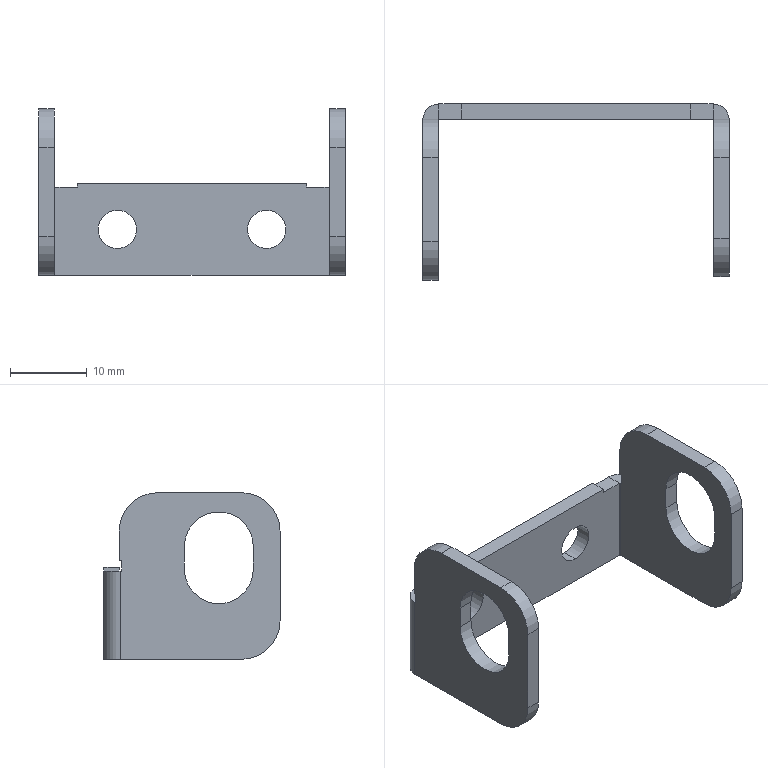Component | SolidWorks | FrontDoorLockRodRetainer-1 | 1 solid | 52 faces | volume 2229 mm3 | plane 34 | cylinder 18 | commonest cylinder face diameters 10 x6 5 x4 9 x4 4.2 x2 0.2 x2